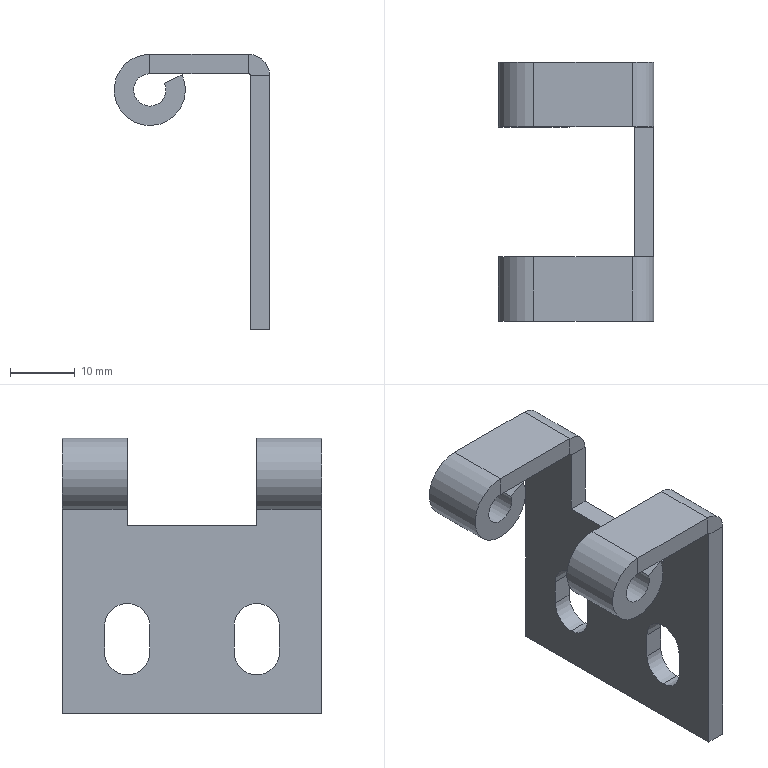Component | SolidWorks | Hinge-2 | 1 solid | 44 faces | volume 6010 mm3 | plane 30 | cylinder 14 | commonest cylinder face diameters 7 x6 6.6 x2 0.6 x2 11 x2 5 x2